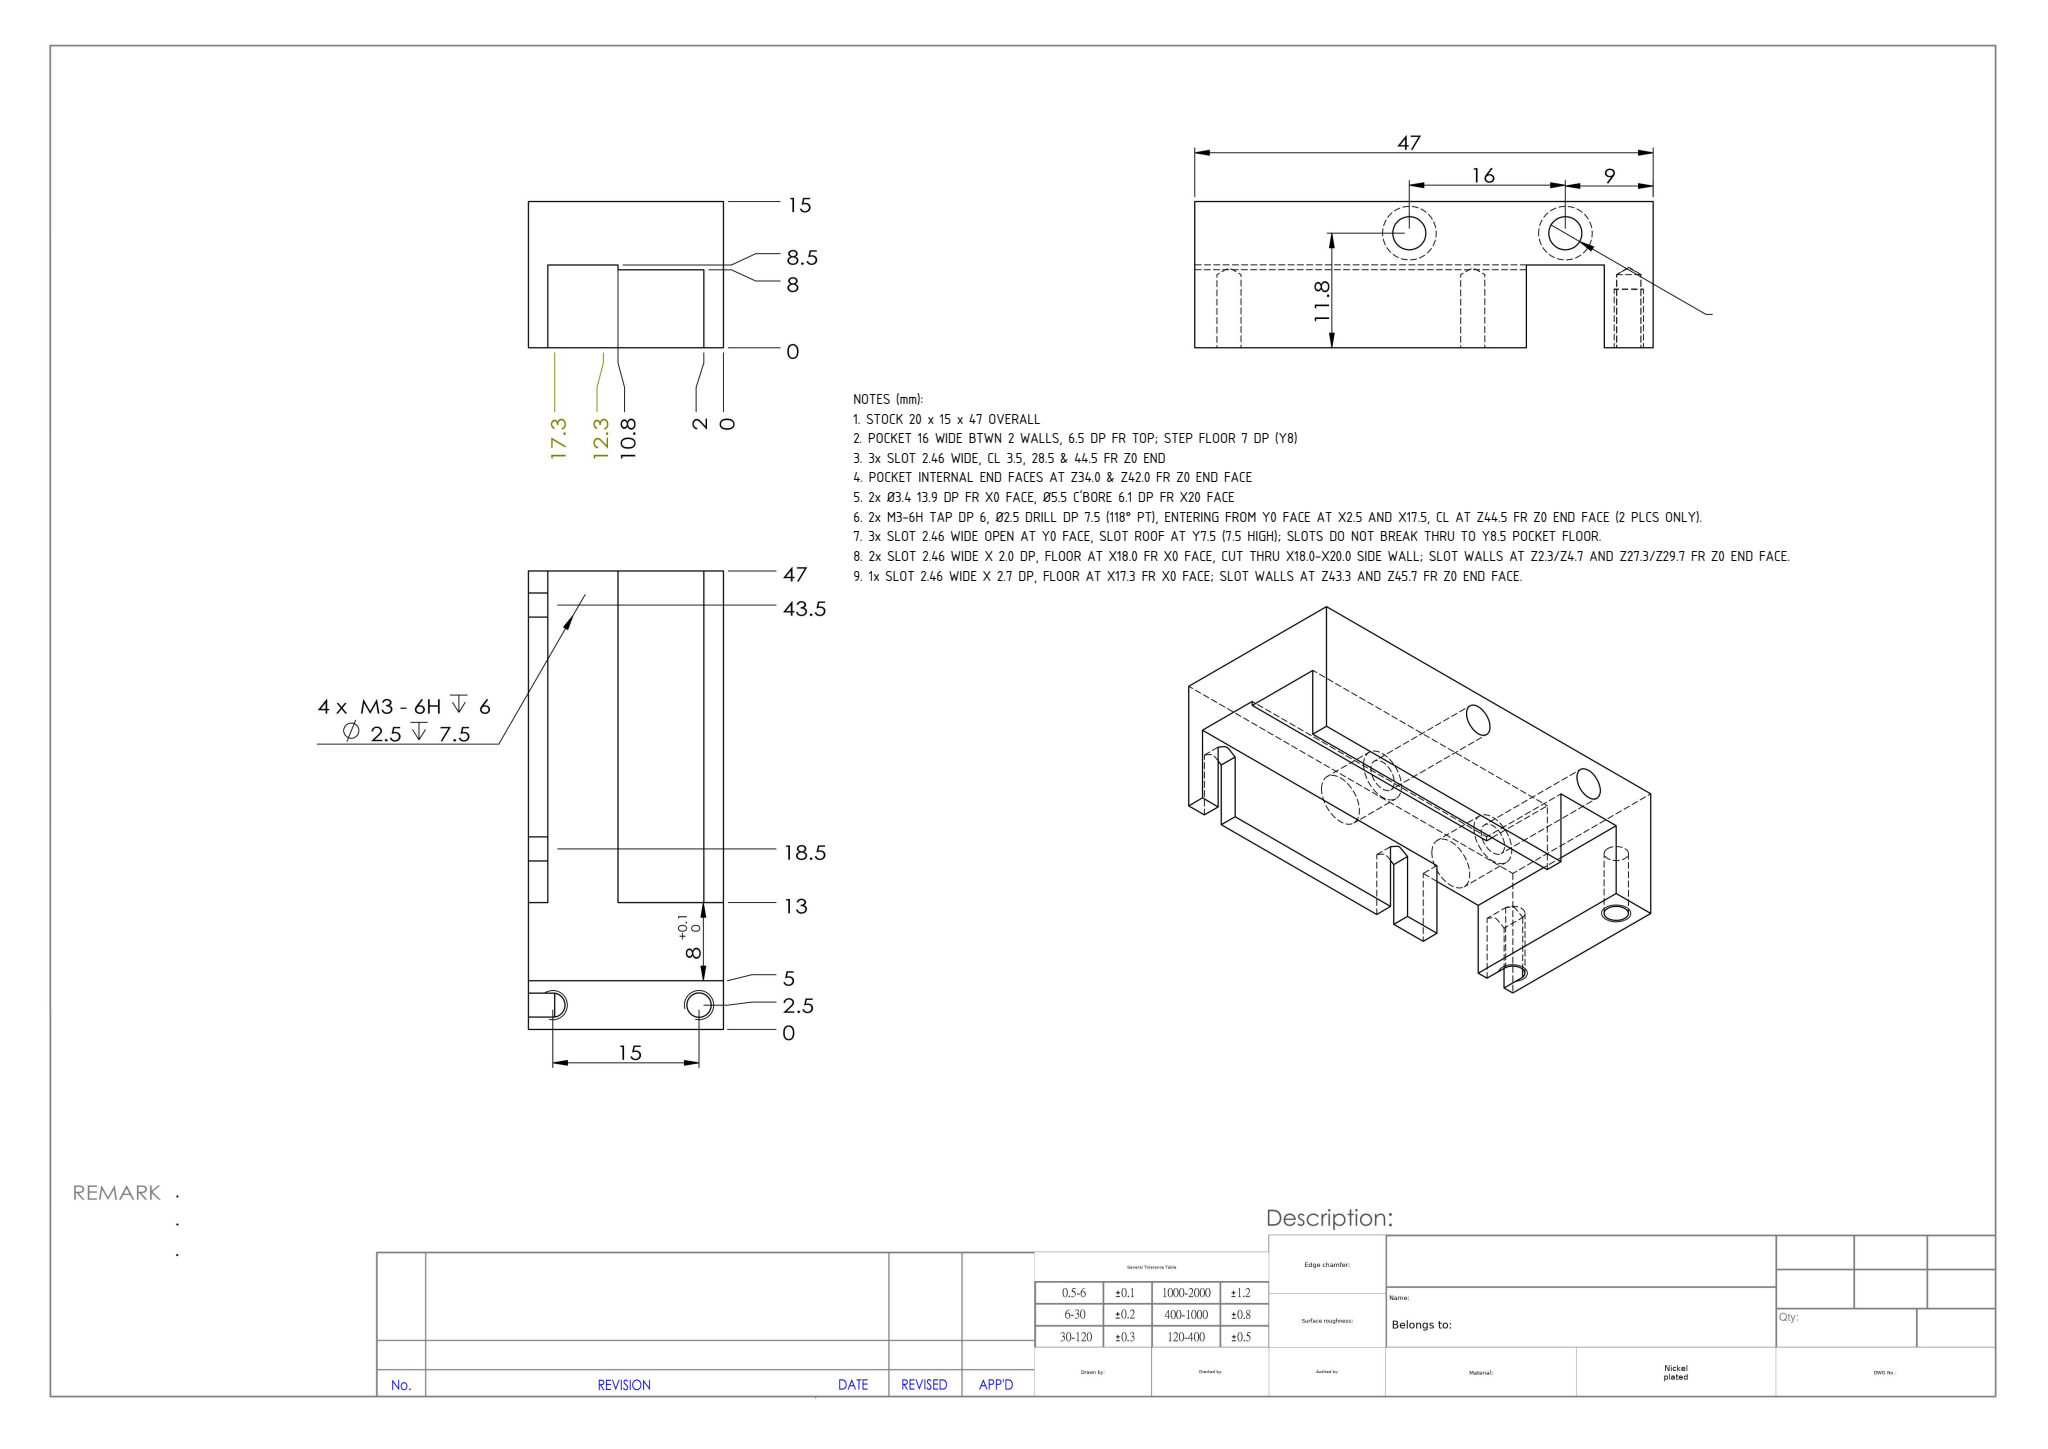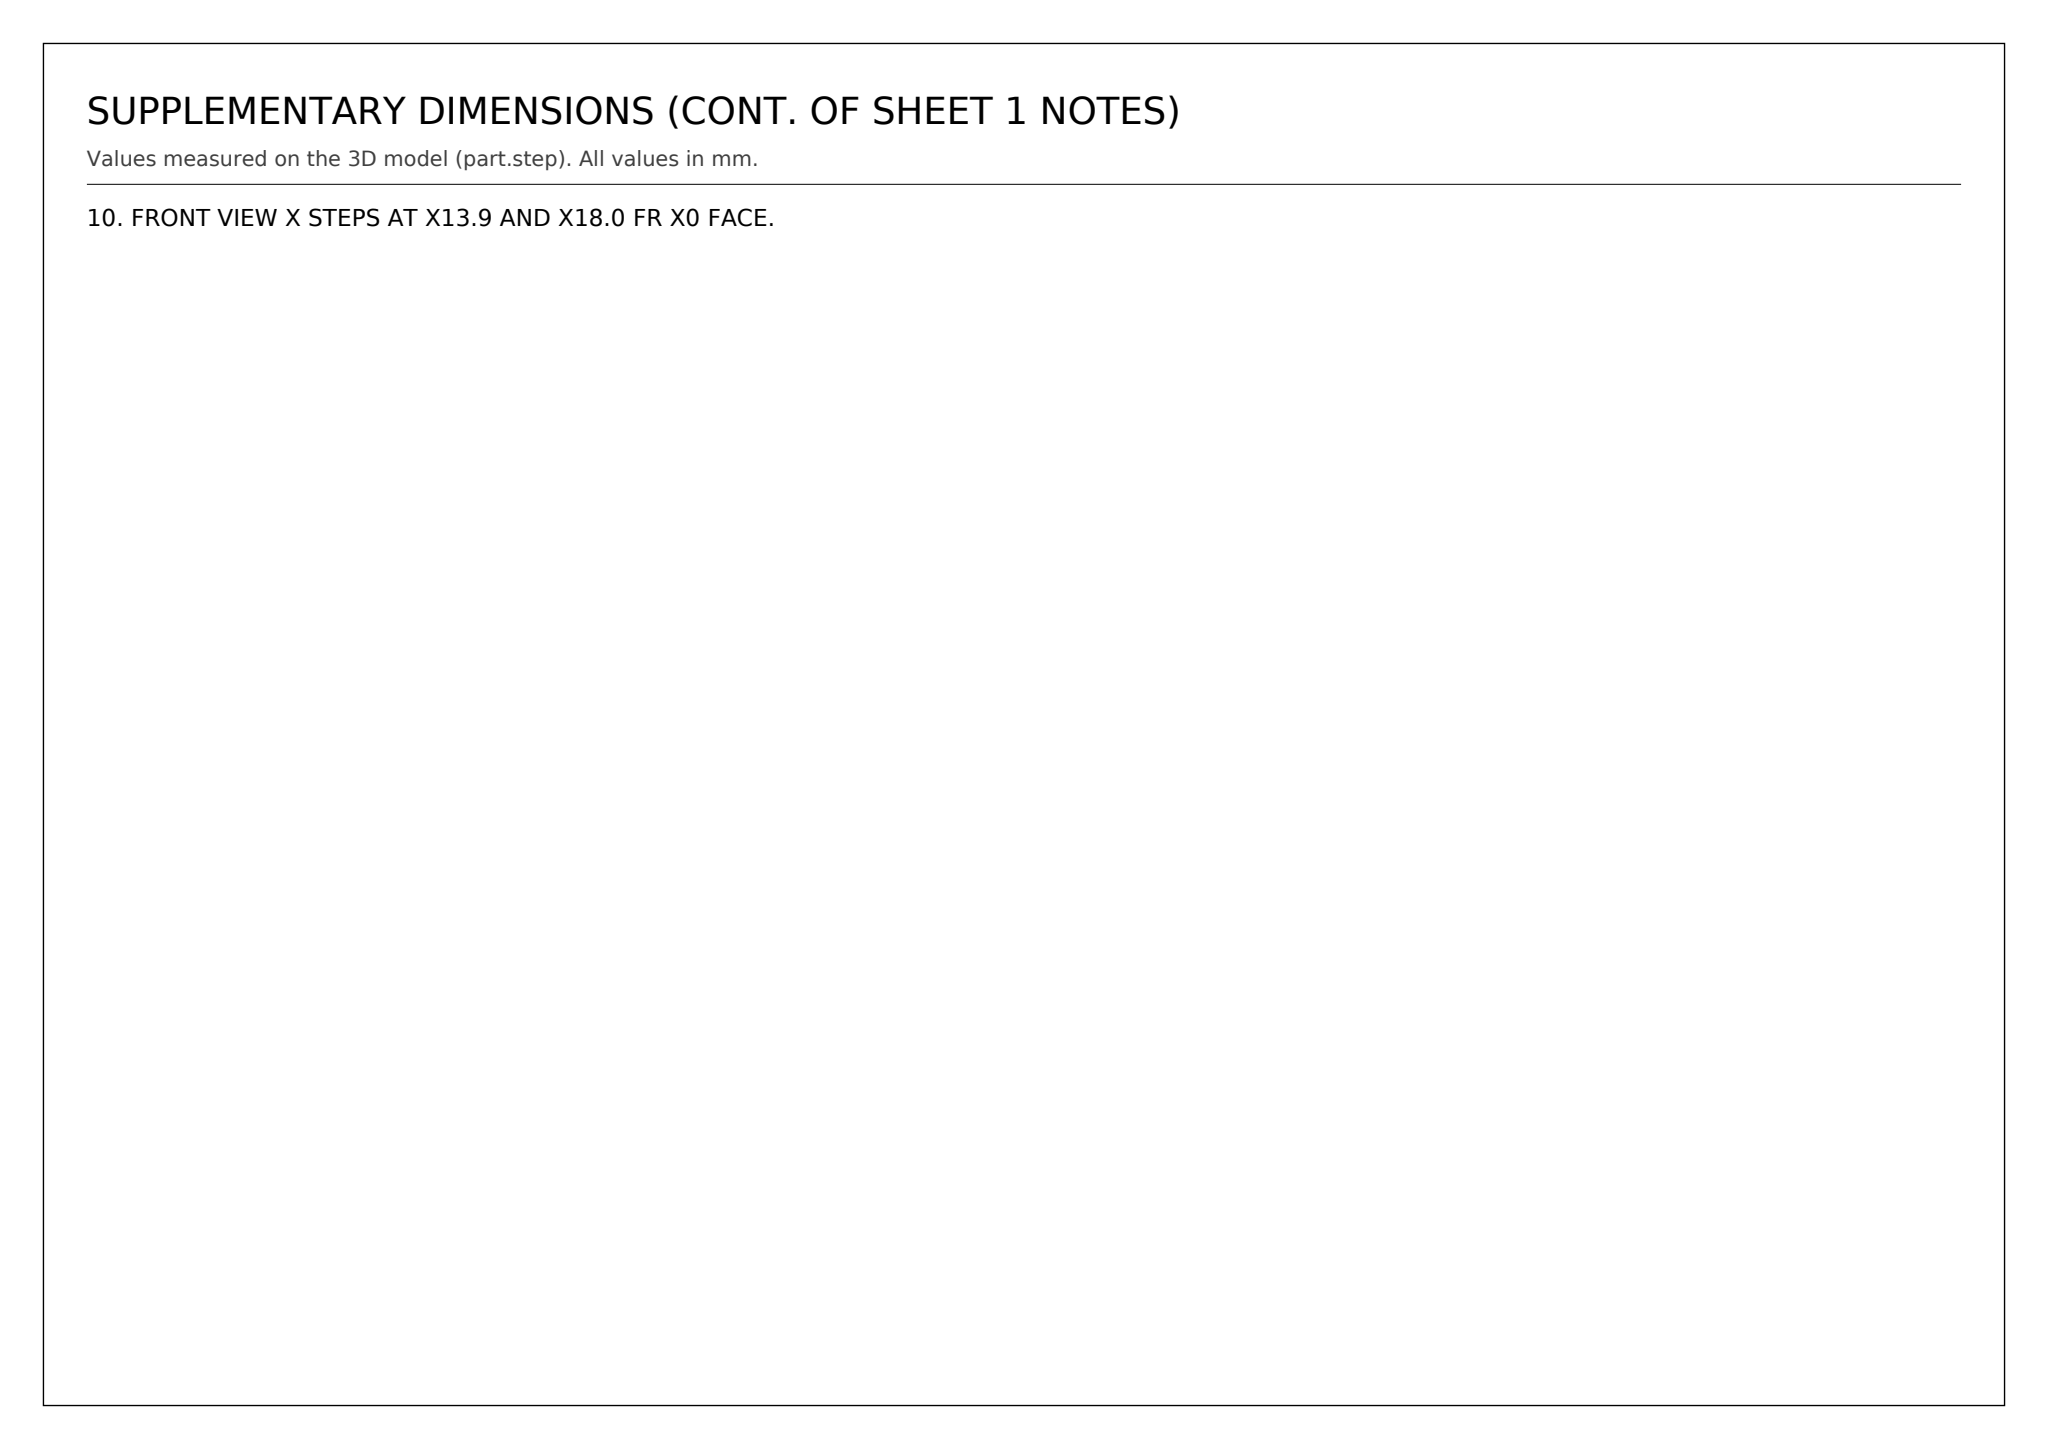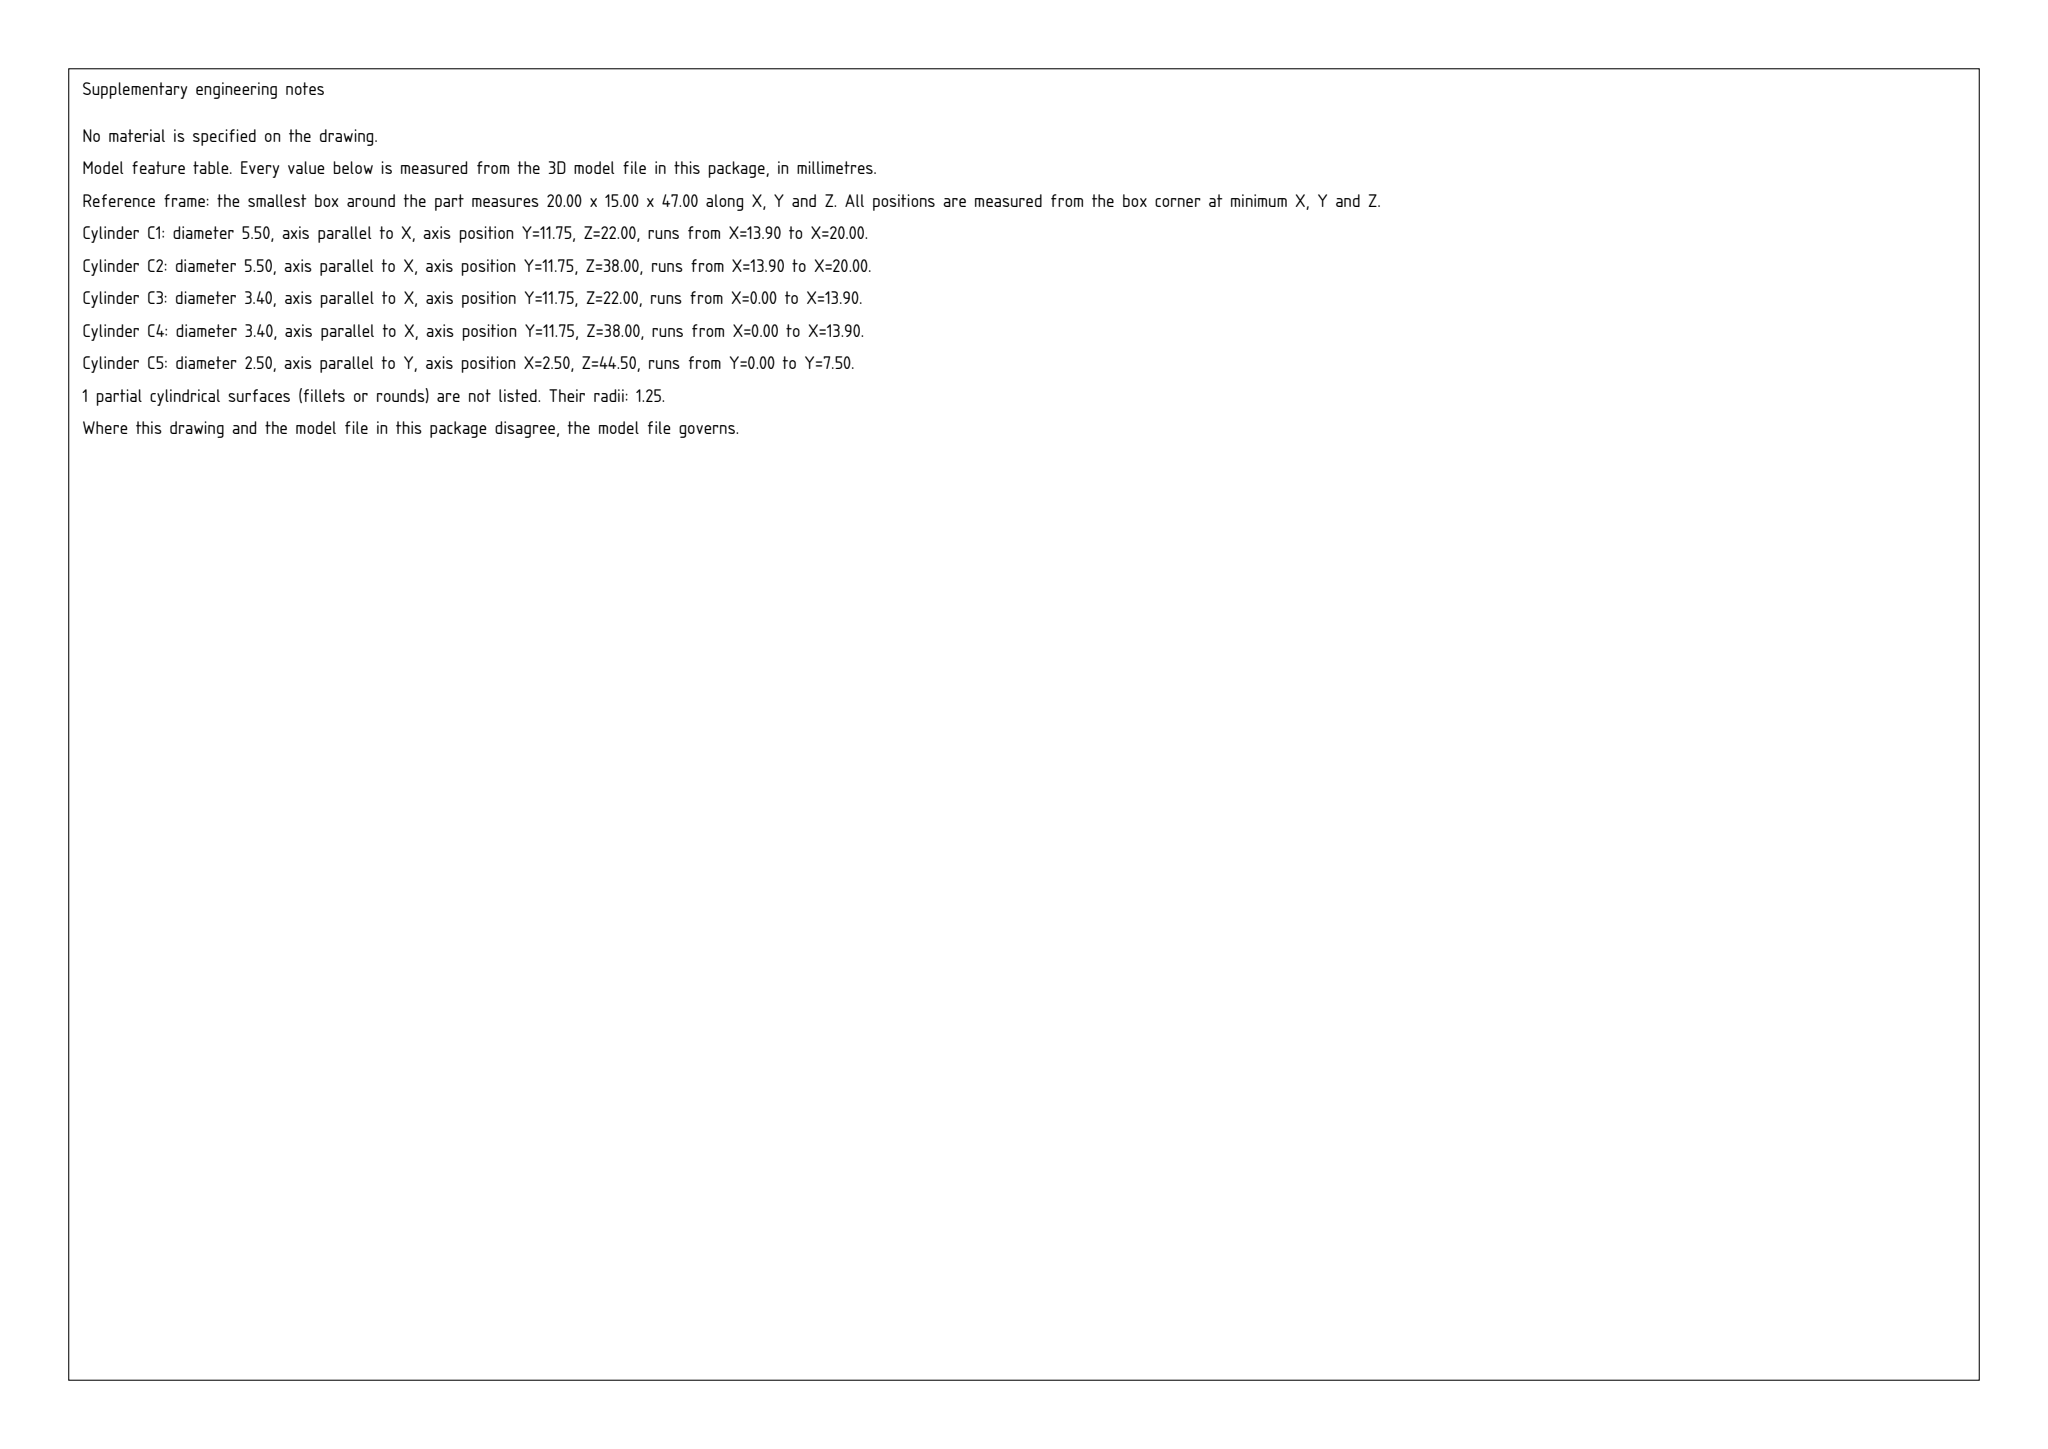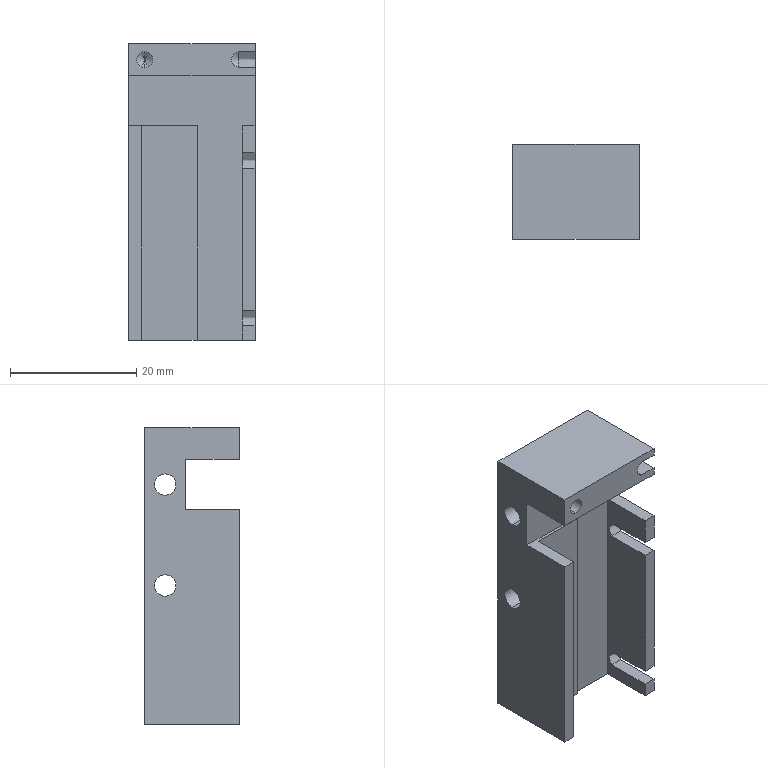Part | SolidWorks | mm | 1 solid | 43 faces | box 20 x 15 x 47 mm | volume 7540 mm3 | plane 26 | cylinder 11 | cone 3 | spline 3 | commonest cylinder face diameters 5.5 x4 3.4 x4 2.5 x3
Drawing notes:
STOCK 20 x 15 x 47 OVERALL | from the solid: bbox_xyz 20 x 15 x 47
POCKET 16 WIDE BTWN 2 WALLS, 6.5 DP FR TOP; STEP FLOOR 7 DP (Y8) | from the solid: x planes 2 & 18 with bbox x=20; y planes 15 top, 8.5 pocket floor, 8 step floor
3x SLOT 2.46 WIDE, CL 3.5, 28.5 & 44.5 FR Z0 END | from the solid: z plane pairs 2.27/4.73, 27.27/29.73, 43.27/45.73 = 2.46 wide, CL 3.5/28.5/44.5
POCKET INTERNAL END FACES AT Z34.0 & Z42.0 FR Z0 END FACE | from the solid: axis_planes z=34.0 (2 faces), z=42.0 (1 face); bbox Z=47
2x Ø3.4 13.9 DP FR X0 FACE, Ø5.5 C'BORE 6.1 DP FR X20 FACE | from the solid: Ø3.4 axis x L13.9 & Ø5.5 axis x L6.1 at z22 & z38; x planes 13.9 & 20
2x M3-6H TAP DP 6, Ø2.5 DRILL DP 7.5 (118° PT), ENTERING FROM Y0 FACE AT X2.5 AND X17.5, CL AT Z44.5 FR Z0 END FACE (2 PLCS ONLY). | from the solid: cylinders Ø2.5 axis y at (x2.5,z44.5) and (x17.5,z44.5), from y0.0 to y7.5; cones 118° ref dia 2.5 at y7.5
3x SLOT 2.46 WIDE OPEN AT Y0 FACE, SLOT ROOF AT Y7.5 (7.5 HIGH); SLOTS DO NOT BREAK THRU TO Y8.5 POCKET FLOOR. | from the solid: slot floor planes z2.3/z4.7/z27.3/z29.7/z43.3/z45.7 all with y extent [0.0, 7.5]
2x SLOT 2.46 WIDE X 2.0 DP, FLOOR AT X18.0 FR X0 FACE, CUT THRU X18.0-X20.0 SIDE WALL; SLOT WALLS AT Z2.3/Z4.7 AND Z27.3/Z29.7 FR Z0 END FACE. | from the solid: x-plane at 18.0 extent y[0,8.5] z[0,34]; z-planes 2.3, 4.7, 27.3, 29.7 extent x[18.0,20.0] y[0,7.5]
1x SLOT 2.46 WIDE X 2.7 DP, FLOOR AT X17.3 FR X0 FACE; SLOT WALLS AT Z43.3 AND Z45.7 FR Z0 END FACE. | from the solid: z-planes 43.3 and 45.7 extent x[17.3,20.0] y[0,7.5]
FRONT VIEW X STEPS AT X13.9 AND X18.0 FR X0 FACE. | from the solid: x-planes at 13.9 (c'bore shoulders) and 18.0 (slot wall face)